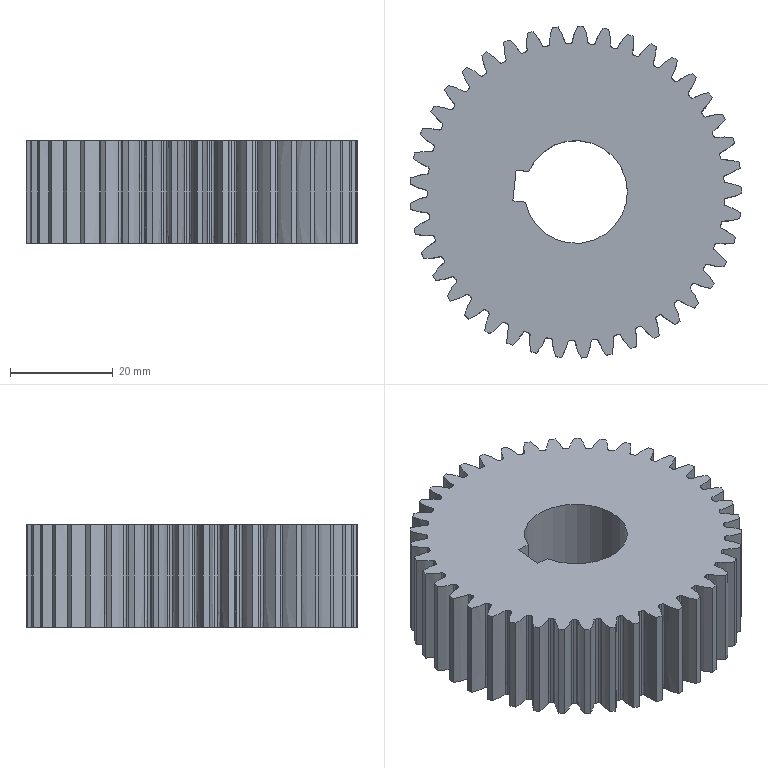Component | NX | DRIVE_GEAR | 1 solid | 252 faces | volume 52420 mm3 | other 205 | cylinder 42 | plane 5 | commonest cylinder face diameters 57.75 x41 20 x1